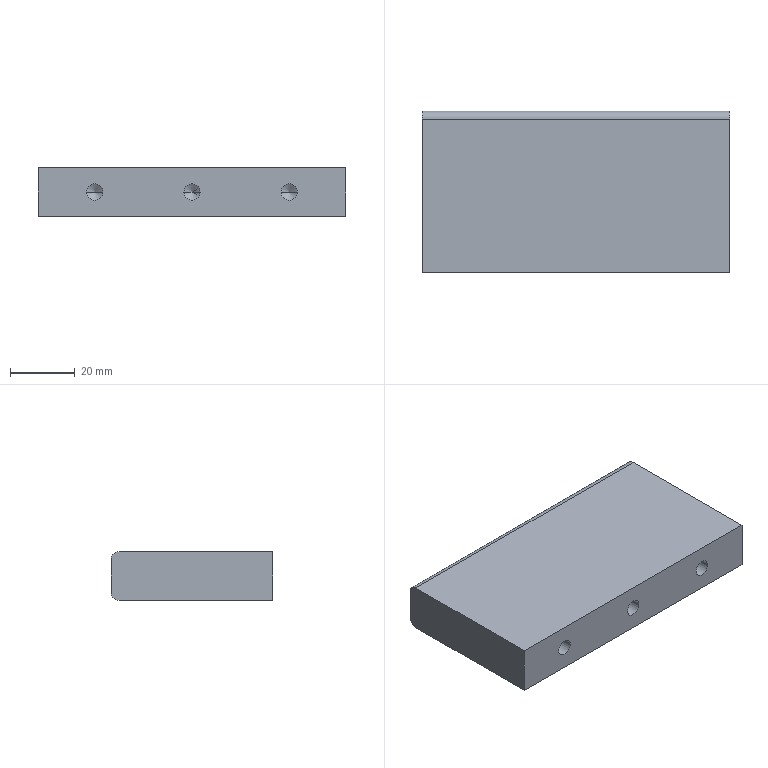Component | SolidWorks | LongSideClampingAssemblyBGeneralAssembly-1_PressBlockB-0510-1 | 1 solid | 20 faces | box 95 x 50 x 15 mm | volume 68763 mm3 | cylinder 8 | cone 6 | plane 6 | commonest cylinder face diameters 5 x8
build123d program:
from build123d import *

# Parameters (mm, degrees)
SKETCH1_W             = 15
SKETCH1_H             = 50
BOSS_EXTRUDE1_DEPTH   = 95
M5_TAPPED_HOLE1_D     = 5
M5_TAPPED_HOLE1_DEPTH = 37.4
M5_TAPPED_HOLE1_TIP   = 1.502
FILLET1_R             = 2.5


with BuildPart() as part:
    # Sketch1 → Boss-Extrude1 (new body)
    with BuildSketch(Plane.XY):
        with Locations((28.929, -13)):
            Rectangle(SKETCH1_W, SKETCH1_H)
    extrude(amount=BOSS_EXTRUDE1_DEPTH)

    # M5 Tapped Hole1
    with Locations(Plane(origin=(0, -38, 0), x_dir=(-1, 0, 0), z_dir=(0, -1, 0))):
        with Locations((-28.929, -47.5), (-28.929, -17.5), (-28.929, -77.5)):
            Hole(M5_TAPPED_HOLE1_D / 2, depth=M5_TAPPED_HOLE1_DEPTH)
            with Locations((0, 0, -(M5_TAPPED_HOLE1_DEPTH + M5_TAPPED_HOLE1_TIP / 2))):  # 118° drill point
                Cone(0, M5_TAPPED_HOLE1_D / 2, M5_TAPPED_HOLE1_TIP, mode=Mode.SUBTRACT)

    # Fillet1
    fillet1_edges = [part.edges().sort_by_distance(p)[0] for p in [
        (21.429, 12, 47.5),
        (36.429, 12, 47.5),
    ]]
    fillet(fillet1_edges, radius=FILLET1_R)


solid = part.part

# Placed as in the assembly
solid = solid.moved(Location((-3168.158, -89.609, 3598.929), (0, 90, 0)))
STEP:
#1=CARTESIAN_POINT('',(-122.762,-3.552,140.551));
#2=VERTEX_POINT('',#1);
#3=CARTESIAN_POINT('',(-122.959,-3.552,140.551));
#4=VERTEX_POINT('',#3);
#5=CARTESIAN_POINT('',(-122.861,-3.552,140.551));
#6=DIRECTION('',(-0.,-1.,0.));
#7=DIRECTION('',(-1.,0.,0.));
#8=AXIS2_PLACEMENT_3D('',#5,#6,#7);
#9=CIRCLE('',#8,0.09843);
#10=EDGE_CURVE('',#2,#4,#9,.T.);
#11=ORIENTED_EDGE('',*,*,#10,.F.);
#12=CARTESIAN_POINT('',(-122.762,-5.024,140.551));
#13=VERTEX_POINT('',#12);
#14=CARTESIAN_POINT('',(-122.762,-5.024,140.551));
#15=DIRECTION('',(-0.,-1.,0.));
#16=VECTOR('',#15,39.37);
#17=LINE('',#14,#16);
#18=EDGE_CURVE('',#2,#13,#17,.T.);
#19=ORIENTED_EDGE('',*,*,#18,.T.);
#20=CARTESIAN_POINT('',(-122.959,-5.024,140.551));
#21=VERTEX_POINT('',#20);
#22=CARTESIAN_POINT('',(-122.861,-5.024,140.551));
#23=DIRECTION('',(-0.,-1.,0.));
#24=DIRECTION('',(-1.,0.,0.));
#25=AXIS2_PLACEMENT_3D('',#22,#23,#24);
#26=CIRCLE('',#25,0.09843);
#27=EDGE_CURVE('',#13,#21,#26,.T.);
#28=ORIENTED_EDGE('',*,*,#27,.T.);
#29=CARTESIAN_POINT('',(-122.959,-5.024,140.551));
#30=DIRECTION('',(-0.,-1.,0.));
#31=VECTOR('',#30,39.37);
#32=LINE('',#29,#31);
#33=EDGE_CURVE('',#4,#21,#32,.T.);
#34=ORIENTED_EDGE('',*,*,#33,.F.);
#35=EDGE_LOOP('',(#11,#19,#28,#34));
#36=FACE_OUTER_BOUND('',#35,.T.);
#37=CARTESIAN_POINT('',(-122.861,-5.024,140.551));
#38=DIRECTION('',(-0.,-1.,0.));
#39=DIRECTION('',(-1.,0.,0.));
#40=AXIS2_PLACEMENT_3D('',#37,#38,#39);
#41=CYLINDRICAL_SURFACE('',#40,0.09843);
#42=ADVANCED_FACE('',(#36),#41,.F.);
#43=CARTESIAN_POINT('',(-122.861,-3.492,140.551));
#44=VERTEX_POINT('',#43);
#45=CARTESIAN_POINT('',(-122.959,-3.552,140.551));
#46=DIRECTION('',(-0.8572,-0.515,-0.));
#47=VECTOR('',#46,39.37);
#48=LINE('',#45,#47);
#49=EDGE_CURVE('',#44,#4,#48,.T.);
#50=ORIENTED_EDGE('',*,*,#49,.F.);
#51=CARTESIAN_POINT('',(-122.762,-3.552,140.551));
#52=DIRECTION('',(0.8572,-0.515,0.));
#53=VECTOR('',#52,39.37);
#54=LINE('',#51,#53);
#55=EDGE_CURVE('',#44,#2,#54,.T.);
#56=ORIENTED_EDGE('',*,*,#55,.T.);
#57=ORIENTED_EDGE('',*,*,#10,.T.);
#58=EDGE_LOOP('',(#50,#56,#57));
#59=FACE_OUTER_BOUND('',#58,.T.);
#60=CARTESIAN_POINT('',(-122.861,-3.552,140.551));
#61=DIRECTION('',(-0.,-1.,0.));
#62=DIRECTION('',(-1.,0.,0.));
#63=AXIS2_PLACEMENT_3D('',#60,#61,#62);
#64=CONICAL_SURFACE('',#63,0.09843,1.03);
#65=ADVANCED_FACE('',(#59),#64,.F.);
#66=CARTESIAN_POINT('',(-123.943,-3.552,140.551));
#67=VERTEX_POINT('',#66);
#68=CARTESIAN_POINT('',(-124.14,-3.552,140.551));
#69=VERTEX_POINT('',#68);
#70=CARTESIAN_POINT('',(-124.042,-3.552,140.551));
#71=DIRECTION('',(-0.,-1.,0.));
#72=DIRECTION('',(-1.,0.,0.));
#73=AXIS2_PLACEMENT_3D('',#70,#71,#72);
#74=CIRCLE('',#73,0.09843);
#75=EDGE_CURVE('',#67,#69,#74,.T.);
#76=ORIENTED_EDGE('',*,*,#75,.F.);
#77=CARTESIAN_POINT('',(-123.943,-5.024,140.551));
#78=VERTEX_POINT('',#77);
#79=CARTESIAN_POINT('',(-123.943,-5.024,140.551));
#80=DIRECTION('',(-0.,-1.,0.));
#81=VECTOR('',#80,39.37);
#82=LINE('',#79,#81);
#83=EDGE_CURVE('',#67,#78,#82,.T.);
#84=ORIENTED_EDGE('',*,*,#83,.T.);
#85=CARTESIAN_POINT('',(-124.14,-5.024,140.551));
#86=VERTEX_POINT('',#85);
#87=CARTESIAN_POINT('',(-124.042,-5.024,140.551));
#88=DIRECTION('',(-0.,-1.,0.));
#89=DIRECTION('',(-1.,0.,0.));
#90=AXIS2_PLACEMENT_3D('',#87,#88,#89);
#91=CIRCLE('',#90,0.09843);
#92=EDGE_CURVE('',#78,#86,#91,.T.);
#93=ORIENTED_EDGE('',*,*,#92,.T.);
#94=CARTESIAN_POINT('',(-124.14,-5.024,140.551));
#95=DIRECTION('',(-0.,-1.,0.));
#96=VECTOR('',#95,39.37);
#97=LINE('',#94,#96);
#98=EDGE_CURVE('',#69,#86,#97,.T.);
#99=ORIENTED_EDGE('',*,*,#98,.F.);
#100=EDGE_LOOP('',(#76,#84,#93,#99));
#101=FACE_OUTER_BOUND('',#100,.T.);
#102=CARTESIAN_POINT('',(-124.042,-5.024,140.551));
#103=DIRECTION('',(-0.,-1.,0.));
#104=DIRECTION('',(-1.,0.,0.));
#105=AXIS2_PLACEMENT_3D('',#102,#103,#104);
#106=CYLINDRICAL_SURFACE('',#105,0.09843);
#107=ADVANCED_FACE('',(#101),#106,.F.);
#108=CARTESIAN_POINT('',(-124.042,-3.492,140.551));
#109=VERTEX_POINT('',#108);
#110=CARTESIAN_POINT('',(-124.14,-3.552,140.551));
#111=DIRECTION('',(-0.8572,-0.515,-0.));
#112=VECTOR('',#111,39.37);
#113=LINE('',#110,#112);
#114=EDGE_CURVE('',#109,#69,#113,.T.);
#115=ORIENTED_EDGE('',*,*,#114,.F.);
#116=CARTESIAN_POINT('',(-123.943,-3.552,140.551));
#117=DIRECTION('',(0.8572,-0.515,0.));
#118=VECTOR('',#117,39.37);
#119=LINE('',#116,#118);
#120=EDGE_CURVE('',#109,#67,#119,.T.);
#121=ORIENTED_EDGE('',*,*,#120,.T.);
#122=ORIENTED_EDGE('',*,*,#75,.T.);
#123=EDGE_LOOP('',(#115,#121,#122));
#124=FACE_OUTER_BOUND('',#123,.T.);
#125=CARTESIAN_POINT('',(-124.042,-3.552,140.551));
#126=DIRECTION('',(-0.,-1.,0.));
#127=DIRECTION('',(-1.,0.,0.));
#128=AXIS2_PLACEMENT_3D('',#125,#126,#127);
#129=CONICAL_SURFACE('',#128,0.09843,1.03);
#130=ADVANCED_FACE('',(#124),#129,.F.);
#131=CARTESIAN_POINT('',(-121.581,-3.552,140.551));
#132=VERTEX_POINT('',#131);
#133=CARTESIAN_POINT('',(-121.778,-3.552,140.551));
#134=VERTEX_POINT('',#133);
#135=CARTESIAN_POINT('',(-121.679,-3.552,140.551));
#136=DIRECTION('',(-0.,-1.,0.));
#137=DIRECTION('',(-1.,0.,0.));
#138=AXIS2_PLACEMENT_3D('',#135,#136,#137);
#139=CIRCLE('',#138,0.09843);
#140=EDGE_CURVE('',#132,#134,#139,.T.);
#141=ORIENTED_EDGE('',*,*,#140,.F.);
#142=CARTESIAN_POINT('',(-121.581,-5.024,140.551));
#143=VERTEX_POINT('',#142);
#144=CARTESIAN_POINT('',(-121.581,-5.024,140.551));
#145=DIRECTION('',(-0.,-1.,0.));
#146=VECTOR('',#145,39.37);
#147=LINE('',#144,#146);
#148=EDGE_CURVE('',#132,#143,#147,.T.);
#149=ORIENTED_EDGE('',*,*,#148,.T.);
#150=CARTESIAN_POINT('',(-121.778,-5.024,140.551));
#151=VERTEX_POINT('',#150);
#152=CARTESIAN_POINT('',(-121.679,-5.024,140.551));
#153=DIRECTION('',(-0.,-1.,0.));
#154=DIRECTION('',(-1.,0.,0.));
#155=AXIS2_PLACEMENT_3D('',#152,#153,#154);
#156=CIRCLE('',#155,0.09843);
#157=EDGE_CURVE('',#143,#151,#156,.T.);
#158=ORIENTED_EDGE('',*,*,#157,.T.);
#159=CARTESIAN_POINT('',(-121.778,-5.024,140.551));
#160=DIRECTION('',(-0.,-1.,0.));
#161=VECTOR('',#160,39.37);
#162=LINE('',#159,#161);
#163=EDGE_CURVE('',#134,#151,#162,.T.);
#164=ORIENTED_EDGE('',*,*,#163,.F.);
#165=EDGE_LOOP('',(#141,#149,#158,#164));
#166=FACE_OUTER_BOUND('',#165,.T.);
#167=CARTESIAN_POINT('',(-121.679,-5.024,140.551));
#168=DIRECTION('',(-0.,-1.,0.));
#169=DIRECTION('',(-1.,0.,0.));
#170=AXIS2_PLACEMENT_3D('',#167,#168,#169);
#171=CYLINDRICAL_SURFACE('',#170,0.09843);
#172=ADVANCED_FACE('',(#166),#171,.F.);
#173=CARTESIAN_POINT('',(-121.679,-3.492,140.551));
#174=VERTEX_POINT('',#173);
#175=CARTESIAN_POINT('',(-121.778,-3.552,140.551));
#176=DIRECTION('',(-0.8572,-0.515,-0.));
#177=VECTOR('',#176,39.37);
#178=LINE('',#175,#177);
#179=EDGE_CURVE('',#174,#134,#178,.T.);
#180=ORIENTED_EDGE('',*,*,#179,.F.);
#181=CARTESIAN_POINT('',(-121.581,-3.552,140.551));
#182=DIRECTION('',(0.8572,-0.515,0.));
#183=VECTOR('',#182,39.37);
#184=LINE('',#181,#183);
#185=EDGE_CURVE('',#174,#132,#184,.T.);
#186=ORIENTED_EDGE('',*,*,#185,.T.);
#187=ORIENTED_EDGE('',*,*,#140,.T.);
#188=EDGE_LOOP('',(#180,#186,#187));
#189=FACE_OUTER_BOUND('',#188,.T.);
#190=CARTESIAN_POINT('',(-121.679,-3.552,140.551));
#191=DIRECTION('',(-0.,-1.,0.));
#192=DIRECTION('',(-1.,0.,0.));
#193=AXIS2_PLACEMENT_3D('',#190,#191,#192);
#194=CONICAL_SURFACE('',#193,0.09843,1.03);
#195=ADVANCED_FACE('',(#189),#194,.F.);
#196=CARTESIAN_POINT('',(-122.861,-5.024,140.551));
#197=DIRECTION('',(-0.,-1.,0.));
#198=DIRECTION('',(-1.,0.,0.));
#199=AXIS2_PLACEMENT_3D('',#196,#197,#198);
#200=CIRCLE('',#199,0.09843);
#201=EDGE_CURVE('',#21,#13,#200,.T.);
#202=ORIENTED_EDGE('',*,*,#201,.F.);
#203=ORIENTED_EDGE('',*,*,#27,.F.);
#204=EDGE_LOOP('',(#202,#203));
#205=FACE_BOUND('',#204,.T.);
#206=CARTESIAN_POINT('',(-124.042,-5.024,140.551));
#207=DIRECTION('',(-0.,-1.,0.));
#208=DIRECTION('',(-1.,0.,0.));
#209=AXIS2_PLACEMENT_3D('',#206,#207,#208);
#210=CIRCLE('',#209,0.09843);
#211=EDGE_CURVE('',#86,#78,#210,.T.);
#212=ORIENTED_EDGE('',*,*,#211,.F.);
#213=ORIENTED_EDGE('',*,*,#92,.F.);
#214=EDGE_LOOP('',(#212,#213));
#215=FACE_BOUND('',#214,.T.);
#216=CARTESIAN_POINT('',(-121.679,-5.024,140.551));
#217=DIRECTION('',(-0.,-1.,0.));
#218=DIRECTION('',(-1.,0.,0.));
#219=AXIS2_PLACEMENT_3D('',#216,#217,#218);
#220=CIRCLE('',#219,0.09843);
#221=EDGE_CURVE('',#151,#143,#220,.T.);
#222=ORIENTED_EDGE('',*,*,#221,.F.);
#223=ORIENTED_EDGE('',*,*,#157,.F.);
#224=EDGE_LOOP('',(#222,#223));
#225=FACE_BOUND('',#224,.T.);
#226=CARTESIAN_POINT('',(-124.731,-5.024,140.846));
#227=VERTEX_POINT('',#226);
#228=CARTESIAN_POINT('',(-124.731,-5.024,140.256));
#229=VERTEX_POINT('',#228);
#230=CARTESIAN_POINT('',(-124.731,-5.024,140.846));
#231=DIRECTION('',(0.,0.,-1.));
#232=VECTOR('',#231,39.37);
#233=LINE('',#230,#232);
#234=EDGE_CURVE('',#227,#229,#233,.T.);
#235=ORIENTED_EDGE('',*,*,#234,.T.);
#236=CARTESIAN_POINT('',(-120.99,-5.024,140.256));
#237=VERTEX_POINT('',#236);
#238=CARTESIAN_POINT('',(-120.99,-5.024,140.256));
#239=DIRECTION('',(-1.,0.,-0.));
#240=VECTOR('',#239,39.37);
#241=LINE('',#238,#240);
#242=EDGE_CURVE('',#237,#229,#241,.T.);
#243=ORIENTED_EDGE('',*,*,#242,.F.);
#244=CARTESIAN_POINT('',(-120.99,-5.024,140.846));
#245=VERTEX_POINT('',#244);
#246=CARTESIAN_POINT('',(-120.99,-5.024,140.846));
#247=DIRECTION('',(0.,0.,-1.));
#248=VECTOR('',#247,39.37);
#249=LINE('',#246,#248);
#250=EDGE_CURVE('',#245,#237,#249,.T.);
#251=ORIENTED_EDGE('',*,*,#250,.F.);
#252=CARTESIAN_POINT('',(-120.99,-5.024,140.846));
#253=DIRECTION('',(-1.,0.,-0.));
#254=VECTOR('',#253,39.37);
#255=LINE('',#252,#254);
#256=EDGE_CURVE('',#245,#227,#255,.T.);
#257=ORIENTED_EDGE('',*,*,#256,.T.);
#258=EDGE_LOOP('',(#235,#243,#251,#257));
#259=FACE_OUTER_BOUND('',#258,.T.);
#260=CARTESIAN_POINT('',(-120.99,-5.024,140.846));
#261=DIRECTION('',(0.,1.,0.));
#262=DIRECTION('',(-0.,-0.,1.));
#263=AXIS2_PLACEMENT_3D('',#260,#261,#262);
#264=PLANE('',#263);
#265=ADVANCED_FACE('',(#205,#215,#225,#259),#264,.F.);
#266=CARTESIAN_POINT('',(-124.731,-3.154,140.256));
#267=VERTEX_POINT('',#266);
#268=CARTESIAN_POINT('',(-124.731,-5.024,140.256));
#269=DIRECTION('',(0.,1.,-0.));
#270=VECTOR('',#269,39.37);
#271=LINE('',#268,#270);
#272=EDGE_CURVE('',#229,#267,#271,.T.);
#273=ORIENTED_EDGE('',*,*,#272,.T.);
#274=CARTESIAN_POINT('',(-120.99,-3.154,140.256));
#275=VERTEX_POINT('',#274);
#276=CARTESIAN_POINT('',(-120.99,-3.154,140.256));
#277=DIRECTION('',(1.,-0.,0.));
#278=VECTOR('',#277,39.37);
#279=LINE('',#276,#278);
#280=EDGE_CURVE('',#267,#275,#279,.T.);
#281=ORIENTED_EDGE('',*,*,#280,.T.);
#282=CARTESIAN_POINT('',(-120.99,-5.024,140.256));
#283=DIRECTION('',(0.,1.,-0.));
#284=VECTOR('',#283,39.37);
#285=LINE('',#282,#284);
#286=EDGE_CURVE('',#237,#275,#285,.T.);
#287=ORIENTED_EDGE('',*,*,#286,.F.);
#288=ORIENTED_EDGE('',*,*,#242,.T.);
#289=EDGE_LOOP('',(#273,#281,#287,#288));
#290=FACE_OUTER_BOUND('',#289,.T.);
#291=CARTESIAN_POINT('',(-120.99,-5.024,140.256));
#292=DIRECTION('',(-0.,0.,1.));
#293=DIRECTION('',(1.,-0.,0.));
#294=AXIS2_PLACEMENT_3D('',#291,#292,#293);
#295=PLANE('',#294);
#296=ADVANCED_FACE('',(#290),#295,.F.);
#297=CARTESIAN_POINT('',(-120.99,-3.055,140.354));
#298=VERTEX_POINT('',#297);
#299=CARTESIAN_POINT('',(-120.99,-3.055,140.748));
#300=VERTEX_POINT('',#299);
#301=CARTESIAN_POINT('',(-120.99,-3.055,140.256));
#302=DIRECTION('',(-0.,-0.,1.));
#303=VECTOR('',#302,39.37);
#304=LINE('',#301,#303);
#305=EDGE_CURVE('',#298,#300,#304,.T.);
#306=ORIENTED_EDGE('',*,*,#305,.F.);
#307=CARTESIAN_POINT('',(-124.731,-3.055,140.354));
#308=VERTEX_POINT('',#307);
#309=CARTESIAN_POINT('',(-120.99,-3.055,140.354));
#310=DIRECTION('',(-1.,0.,-0.));
#311=VECTOR('',#310,39.37);
#312=LINE('',#309,#311);
#313=EDGE_CURVE('',#298,#308,#312,.T.);
#314=ORIENTED_EDGE('',*,*,#313,.T.);
#315=CARTESIAN_POINT('',(-124.731,-3.055,140.748));
#316=VERTEX_POINT('',#315);
#317=CARTESIAN_POINT('',(-124.731,-3.055,140.256));
#318=DIRECTION('',(-0.,-0.,1.));
#319=VECTOR('',#318,39.37);
#320=LINE('',#317,#319);
#321=EDGE_CURVE('',#308,#316,#320,.T.);
#322=ORIENTED_EDGE('',*,*,#321,.T.);
#323=CARTESIAN_POINT('',(-120.99,-3.055,140.748));
#324=DIRECTION('',(1.,-0.,0.));
#325=VECTOR('',#324,39.37);
#326=LINE('',#323,#325);
#327=EDGE_CURVE('',#316,#300,#326,.T.);
#328=ORIENTED_EDGE('',*,*,#327,.T.);
#329=EDGE_LOOP('',(#306,#314,#322,#328));
#330=FACE_OUTER_BOUND('',#329,.T.);
#331=CARTESIAN_POINT('',(-120.99,-3.055,140.256));
#332=DIRECTION('',(-0.,-1.,-0.));
#333=DIRECTION('',(0.,0.,-1.));
#334=AXIS2_PLACEMENT_3D('',#331,#332,#333);
#335=PLANE('',#334);
#336=ADVANCED_FACE('',(#330),#335,.F.);
#337=CARTESIAN_POINT('',(-120.99,-3.154,140.846));
#338=VERTEX_POINT('',#337);
#339=CARTESIAN_POINT('',(-120.99,-3.055,140.846));
#340=DIRECTION('',(-0.,-1.,-0.));
#341=VECTOR('',#340,39.37);
#342=LINE('',#339,#341);
#343=EDGE_CURVE('',#338,#245,#342,.T.);
#344=ORIENTED_EDGE('',*,*,#343,.F.);
#345=CARTESIAN_POINT('',(-124.731,-3.154,140.846));
#346=VERTEX_POINT('',#345);
#347=CARTESIAN_POINT('',(-120.99,-3.154,140.846));
#348=DIRECTION('',(-1.,0.,-0.));
#349=VECTOR('',#348,39.37);
#350=LINE('',#347,#349);
#351=EDGE_CURVE('',#338,#346,#350,.T.);
#352=ORIENTED_EDGE('',*,*,#351,.T.);
#353=CARTESIAN_POINT('',(-124.731,-3.055,140.846));
#354=DIRECTION('',(-0.,-1.,-0.));
#355=VECTOR('',#354,39.37);
#356=LINE('',#353,#355);
#357=EDGE_CURVE('',#346,#227,#356,.T.);
#358=ORIENTED_EDGE('',*,*,#357,.T.);
#359=ORIENTED_EDGE('',*,*,#256,.F.);
#360=EDGE_LOOP('',(#344,#352,#358,#359));
#361=FACE_OUTER_BOUND('',#360,.T.);
#362=CARTESIAN_POINT('',(-120.99,-3.055,140.846));
#363=DIRECTION('',(0.,0.,-1.));
#364=DIRECTION('',(0.,1.,0.));
#365=AXIS2_PLACEMENT_3D('',#362,#363,#364);
#366=PLANE('',#365);
#367=ADVANCED_FACE('',(#361),#366,.F.);
#368=ORIENTED_EDGE('',*,*,#286,.T.);
#369=CARTESIAN_POINT('',(-120.99,-3.154,140.354));
#370=DIRECTION('',(1.,-0.,0.));
#371=DIRECTION('',(0.,0.,-1.));
#372=AXIS2_PLACEMENT_3D('',#369,#370,#371);
#373=CIRCLE('',#372,0.09843);
#374=EDGE_CURVE('',#275,#298,#373,.T.);
#375=ORIENTED_EDGE('',*,*,#374,.T.);
#376=ORIENTED_EDGE('',*,*,#305,.T.);
#377=CARTESIAN_POINT('',(-120.99,-3.154,140.748));
#378=DIRECTION('',(1.,-0.,0.));
#379=DIRECTION('',(0.,0.,-1.));
#380=AXIS2_PLACEMENT_3D('',#377,#378,#379);
#381=CIRCLE('',#380,0.09843);
#382=EDGE_CURVE('',#300,#338,#381,.T.);
#383=ORIENTED_EDGE('',*,*,#382,.T.);
#384=ORIENTED_EDGE('',*,*,#343,.T.);
#385=ORIENTED_EDGE('',*,*,#250,.T.);
#386=EDGE_LOOP('',(#368,#375,#376,#383,#384,#385));
#387=FACE_OUTER_BOUND('',#386,.T.);
#388=CARTESIAN_POINT('',(-120.99,-3.528,141.69));
#389=DIRECTION('',(1.,-0.,0.));
#390=DIRECTION('',(0.,-0.,-1.));
#391=AXIS2_PLACEMENT_3D('',#388,#389,#390);
#392=PLANE('',#391);
#393=ADVANCED_FACE('',(#387),#392,.T.);
#394=ORIENTED_EDGE('',*,*,#321,.F.);
#395=CARTESIAN_POINT('',(-124.731,-3.154,140.354));
#396=DIRECTION('',(-1.,0.,-0.));
#397=DIRECTION('',(0.,0.,-1.));
#398=AXIS2_PLACEMENT_3D('',#395,#396,#397);
#399=CIRCLE('',#398,0.09843);
#400=EDGE_CURVE('',#308,#267,#399,.T.);
#401=ORIENTED_EDGE('',*,*,#400,.T.);
#402=ORIENTED_EDGE('',*,*,#272,.F.);
#403=ORIENTED_EDGE('',*,*,#234,.F.);
#404=ORIENTED_EDGE('',*,*,#357,.F.);
#405=CARTESIAN_POINT('',(-124.731,-3.154,140.748));
#406=DIRECTION('',(-1.,0.,-0.));
#407=DIRECTION('',(0.,0.,-1.));
#408=AXIS2_PLACEMENT_3D('',#405,#406,#407);
#409=CIRCLE('',#408,0.09843);
#410=EDGE_CURVE('',#346,#316,#409,.T.);
#411=ORIENTED_EDGE('',*,*,#410,.T.);
#412=EDGE_LOOP('',(#394,#401,#402,#403,#404,#411));
#413=FACE_OUTER_BOUND('',#412,.T.);
#414=CARTESIAN_POINT('',(-124.731,-3.528,141.69));
#415=DIRECTION('',(1.,-0.,0.));
#416=DIRECTION('',(0.,-0.,-1.));
#417=AXIS2_PLACEMENT_3D('',#414,#415,#416);
#418=PLANE('',#417);
#419=ADVANCED_FACE('',(#413),#418,.F.);
#420=ORIENTED_EDGE('',*,*,#185,.F.);
#421=ORIENTED_EDGE('',*,*,#179,.T.);
#422=CARTESIAN_POINT('',(-121.679,-3.552,140.551));
#423=DIRECTION('',(-0.,-1.,0.));
#424=DIRECTION('',(-1.,0.,0.));
#425=AXIS2_PLACEMENT_3D('',#422,#423,#424);
#426=CIRCLE('',#425,0.09843);
#427=EDGE_CURVE('',#134,#132,#426,.T.);
#428=ORIENTED_EDGE('',*,*,#427,.T.);
#429=EDGE_LOOP('',(#420,#421,#428));
#430=FACE_OUTER_BOUND('',#429,.T.);
#431=CARTESIAN_POINT('',(-121.679,-3.552,140.551));
#432=DIRECTION('',(-0.,-1.,0.));
#433=DIRECTION('',(-1.,0.,0.));
#434=AXIS2_PLACEMENT_3D('',#431,#432,#433);
#435=CONICAL_SURFACE('',#434,0.09843,1.03);
#436=ADVANCED_FACE('',(#430),#435,.F.);
#437=ORIENTED_EDGE('',*,*,#148,.F.);
#438=ORIENTED_EDGE('',*,*,#427,.F.);
#439=ORIENTED_EDGE('',*,*,#163,.T.);
#440=ORIENTED_EDGE('',*,*,#221,.T.);
#441=EDGE_LOOP('',(#437,#438,#439,#440));
#442=FACE_OUTER_BOUND('',#441,.T.);
#443=CARTESIAN_POINT('',(-121.679,-5.024,140.551));
#444=DIRECTION('',(-0.,-1.,0.));
#445=DIRECTION('',(-1.,0.,0.));
#446=AXIS2_PLACEMENT_3D('',#443,#444,#445);
#447=CYLINDRICAL_SURFACE('',#446,0.09843);
#448=ADVANCED_FACE('',(#442),#447,.F.);
#449=ORIENTED_EDGE('',*,*,#120,.F.);
#450=ORIENTED_EDGE('',*,*,#114,.T.);
#451=CARTESIAN_POINT('',(-124.042,-3.552,140.551));
#452=DIRECTION('',(-0.,-1.,0.));
#453=DIRECTION('',(-1.,0.,0.));
#454=AXIS2_PLACEMENT_3D('',#451,#452,#453);
#455=CIRCLE('',#454,0.09843);
#456=EDGE_CURVE('',#69,#67,#455,.T.);
#457=ORIENTED_EDGE('',*,*,#456,.T.);
#458=EDGE_LOOP('',(#449,#450,#457));
#459=FACE_OUTER_BOUND('',#458,.T.);
#460=CARTESIAN_POINT('',(-124.042,-3.552,140.551));
#461=DIRECTION('',(-0.,-1.,0.));
#462=DIRECTION('',(-1.,0.,0.));
#463=AXIS2_PLACEMENT_3D('',#460,#461,#462);
#464=CONICAL_SURFACE('',#463,0.09843,1.03);
#465=ADVANCED_FACE('',(#459),#464,.F.);
#466=ORIENTED_EDGE('',*,*,#83,.F.);
#467=ORIENTED_EDGE('',*,*,#456,.F.);
#468=ORIENTED_EDGE('',*,*,#98,.T.);
#469=ORIENTED_EDGE('',*,*,#211,.T.);
#470=EDGE_LOOP('',(#466,#467,#468,#469));
#471=FACE_OUTER_BOUND('',#470,.T.);
#472=CARTESIAN_POINT('',(-124.042,-5.024,140.551));
#473=DIRECTION('',(-0.,-1.,0.));
#474=DIRECTION('',(-1.,0.,0.));
#475=AXIS2_PLACEMENT_3D('',#472,#473,#474);
#476=CYLINDRICAL_SURFACE('',#475,0.09843);
#477=ADVANCED_FACE('',(#471),#476,.F.);
#478=ORIENTED_EDGE('',*,*,#55,.F.);
#479=ORIENTED_EDGE('',*,*,#49,.T.);
#480=CARTESIAN_POINT('',(-122.861,-3.552,140.551));
#481=DIRECTION('',(-0.,-1.,0.));
#482=DIRECTION('',(-1.,0.,0.));
#483=AXIS2_PLACEMENT_3D('',#480,#481,#482);
#484=CIRCLE('',#483,0.09843);
#485=EDGE_CURVE('',#4,#2,#484,.T.);
#486=ORIENTED_EDGE('',*,*,#485,.T.);
#487=EDGE_LOOP('',(#478,#479,#486));
#488=FACE_OUTER_BOUND('',#487,.T.);
#489=CARTESIAN_POINT('',(-122.861,-3.552,140.551));
#490=DIRECTION('',(-0.,-1.,0.));
#491=DIRECTION('',(-1.,0.,0.));
#492=AXIS2_PLACEMENT_3D('',#489,#490,#491);
#493=CONICAL_SURFACE('',#492,0.09843,1.03);
#494=ADVANCED_FACE('',(#488),#493,.F.);
#495=ORIENTED_EDGE('',*,*,#18,.F.);
#496=ORIENTED_EDGE('',*,*,#485,.F.);
#497=ORIENTED_EDGE('',*,*,#33,.T.);
#498=ORIENTED_EDGE('',*,*,#201,.T.);
#499=EDGE_LOOP('',(#495,#496,#497,#498));
#500=FACE_OUTER_BOUND('',#499,.T.);
#501=CARTESIAN_POINT('',(-122.861,-5.024,140.551));
#502=DIRECTION('',(-0.,-1.,0.));
#503=DIRECTION('',(-1.,0.,0.));
#504=AXIS2_PLACEMENT_3D('',#501,#502,#503);
#505=CYLINDRICAL_SURFACE('',#504,0.09843);
#506=ADVANCED_FACE('',(#500),#505,.F.);
#507=ORIENTED_EDGE('',*,*,#374,.F.);
#508=ORIENTED_EDGE('',*,*,#280,.F.);
#509=ORIENTED_EDGE('',*,*,#400,.F.);
#510=ORIENTED_EDGE('',*,*,#313,.F.);
#511=EDGE_LOOP('',(#507,#508,#509,#510));
#512=FACE_OUTER_BOUND('',#511,.T.);
#513=CARTESIAN_POINT('',(-120.99,-3.154,140.354));
#514=DIRECTION('',(-1.,0.,-0.));
#515=DIRECTION('',(0.,0.,1.));
#516=AXIS2_PLACEMENT_3D('',#513,#514,#515);
#517=CYLINDRICAL_SURFACE('',#516,0.09843);
#518=ADVANCED_FACE('',(#512),#517,.T.);
#519=ORIENTED_EDGE('',*,*,#382,.F.);
#520=ORIENTED_EDGE('',*,*,#327,.F.);
#521=ORIENTED_EDGE('',*,*,#410,.F.);
#522=ORIENTED_EDGE('',*,*,#351,.F.);
#523=EDGE_LOOP('',(#519,#520,#521,#522));
#524=FACE_OUTER_BOUND('',#523,.T.);
#525=CARTESIAN_POINT('',(-120.99,-3.154,140.748));
#526=DIRECTION('',(-1.,0.,-0.));
#527=DIRECTION('',(0.,0.,1.));
#528=AXIS2_PLACEMENT_3D('',#525,#526,#527);
#529=CYLINDRICAL_SURFACE('',#528,0.09843);
#530=ADVANCED_FACE('',(#524),#529,.T.);
#531=CLOSED_SHELL('',(#42,#65,#107,#130,#172,#195,#265,#296,#336,#367,#393,#419,#436,#448,#465,#477,#494,#506,#518,#530));
#532=MANIFOLD_SOLID_BREP('',#531);
#533=CARTESIAN_POINT('',(0.,0.,0.));
#534=DIRECTION('',(0.,0.,1.));
#535=DIRECTION('',(1.,0.,0.));
#536=AXIS2_PLACEMENT_3D('',#533,#534,#535);
#537=(LENGTH_UNIT()NAMED_UNIT(*)SI_UNIT($,.METRE.));
#538=LENGTH_MEASURE_WITH_UNIT(LENGTH_MEASURE(0.0254),#537);
#539=DIMENSIONAL_EXPONENTS(1.,0.,0.,0.,0.,0.,0.);
#540=(CONVERSION_BASED_UNIT('',#538)LENGTH_UNIT()NAMED_UNIT(#539));
#541=UNCERTAINTY_MEASURE_WITH_UNIT(LENGTH_MEASURE(0.00001),#540,'','');
#542=(NAMED_UNIT(*)PLANE_ANGLE_UNIT()SI_UNIT($,.RADIAN.));
#543=(NAMED_UNIT(*)SI_UNIT($,.STERADIAN.)SOLID_ANGLE_UNIT());
#544=(GEOMETRIC_REPRESENTATION_CONTEXT(3)GLOBAL_UNCERTAINTY_ASSIGNED_CONTEXT((#541))GLOBAL_UNIT_ASSIGNED_CONTEXT((#540,#542,#543))REPRESENTATION_CONTEXT('',''));
#545=ADVANCED_BREP_SHAPE_REPRESENTATION('',(#532,#536),#544);
#546=COLOUR_RGB('',0.7922,0.8196,0.9333);
#547=FILL_AREA_STYLE_COLOUR('',#546);
#548=FILL_AREA_STYLE('',(#547));
#549=SURFACE_STYLE_FILL_AREA(#548);
#550=SURFACE_SIDE_STYLE('',(#549));
#551=SURFACE_STYLE_USAGE(.BOTH.,#550);
#552=PRESENTATION_STYLE_ASSIGNMENT((#551));
#553=STYLED_ITEM('',(#552),#532);
#554=PRESENTATION_LAYER_ASSIGNMENT('','',(#553));
#555=(LENGTH_UNIT()NAMED_UNIT(*)SI_UNIT($,.METRE.));
#556=LENGTH_MEASURE_WITH_UNIT(LENGTH_MEASURE(0.0254),#555);
#557=DIMENSIONAL_EXPONENTS(1.,0.,0.,0.,0.,0.,0.);
#558=(CONVERSION_BASED_UNIT('',#556)LENGTH_UNIT()NAMED_UNIT(#557));
#559=UNCERTAINTY_MEASURE_WITH_UNIT(LENGTH_MEASURE(0.00001),#558,'','');
#560=(NAMED_UNIT(*)PLANE_ANGLE_UNIT()SI_UNIT($,.RADIAN.));
#561=(NAMED_UNIT(*)SI_UNIT($,.STERADIAN.)SOLID_ANGLE_UNIT());
#562=(GEOMETRIC_REPRESENTATION_CONTEXT(3)GLOBAL_UNCERTAINTY_ASSIGNED_CONTEXT((#559))GLOBAL_UNIT_ASSIGNED_CONTEXT((#558,#560,#561))REPRESENTATION_CONTEXT('',''));
#563=MECHANICAL_DESIGN_GEOMETRIC_PRESENTATION_REPRESENTATION('',(#553),#562);